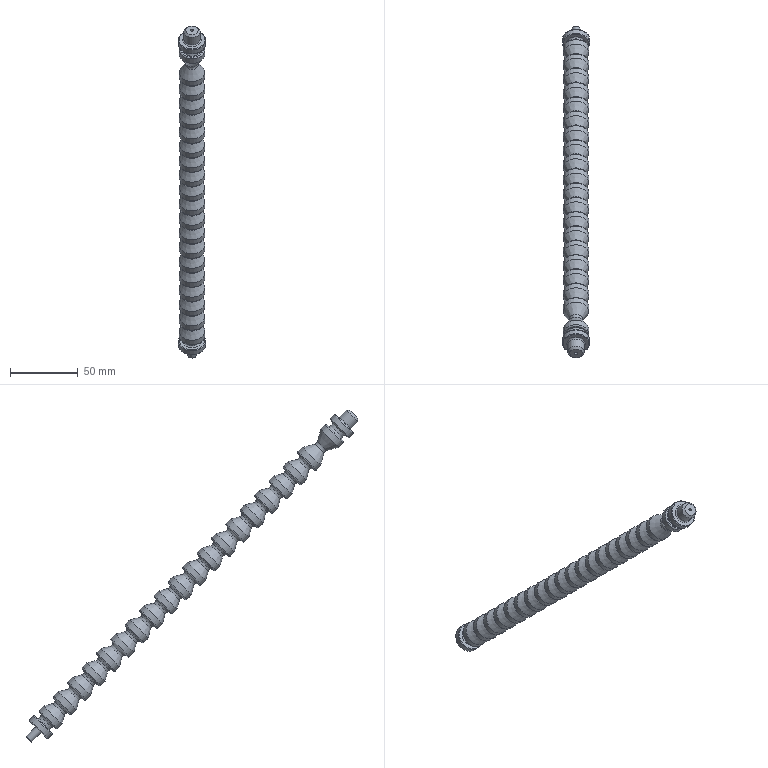Component | NX | UNIVERSAL_JOINT_TUBE | 21 solids | 260 faces | volume 63165 mm3 | cylinder 85 | torus 48 | plane 46 | cone 41 | sphere 40 | commonest cylinder face diameters 2 x21 12 x21 15 x20 19 x20 20 x2 6 x1